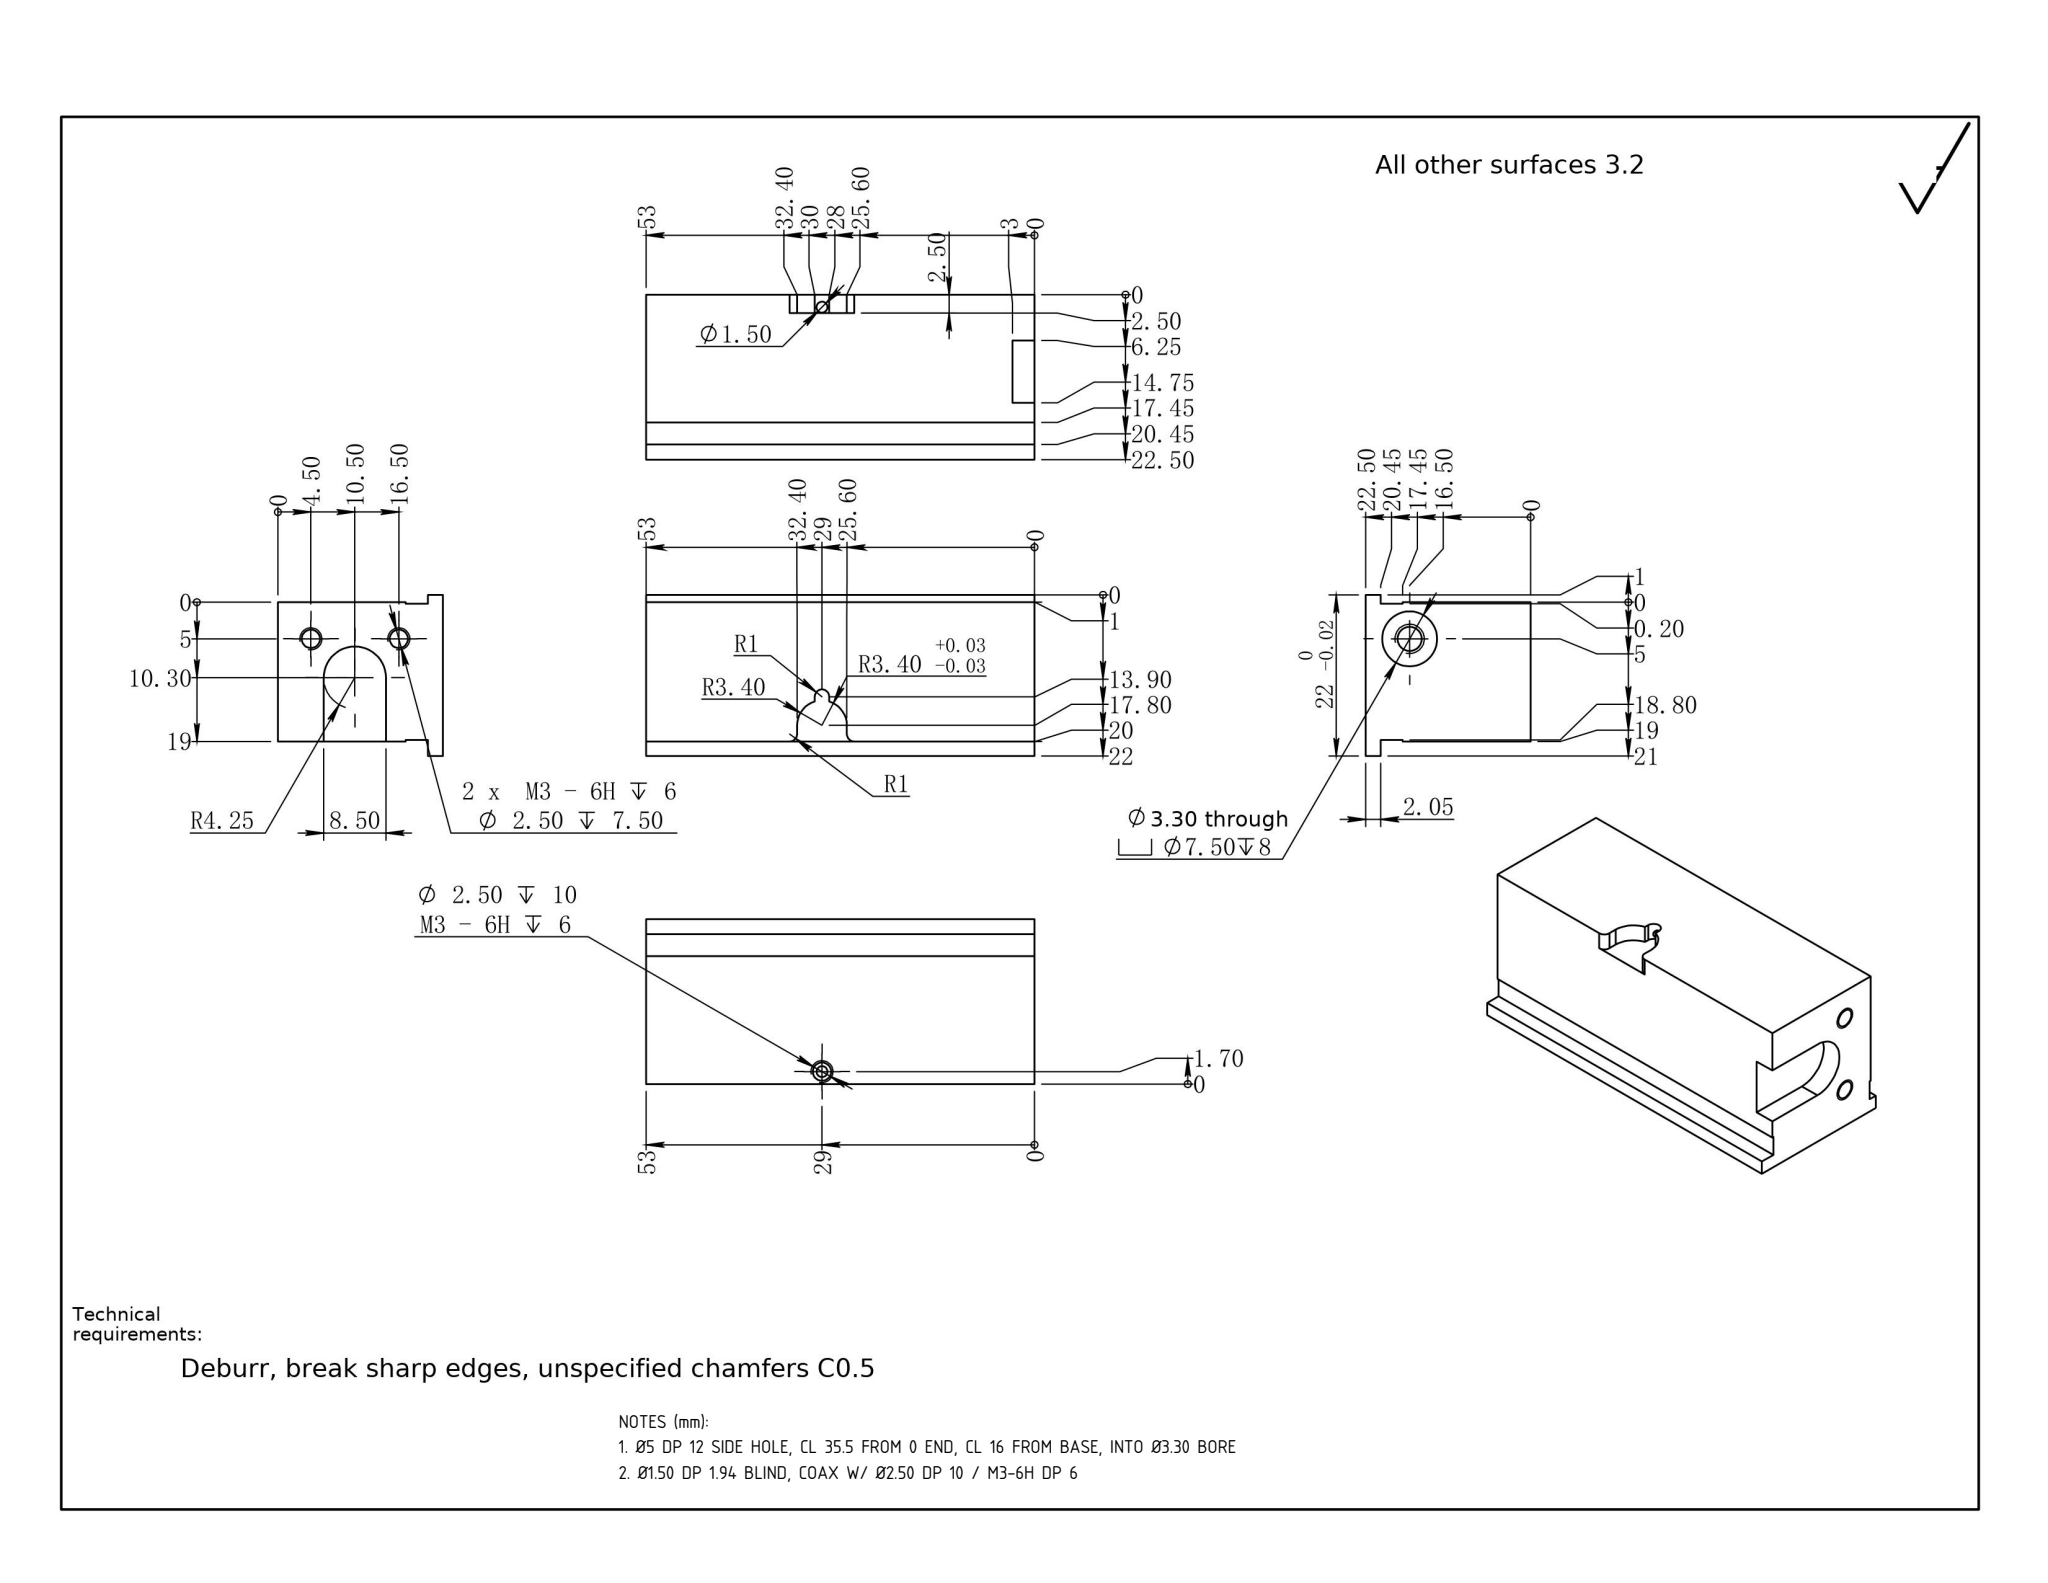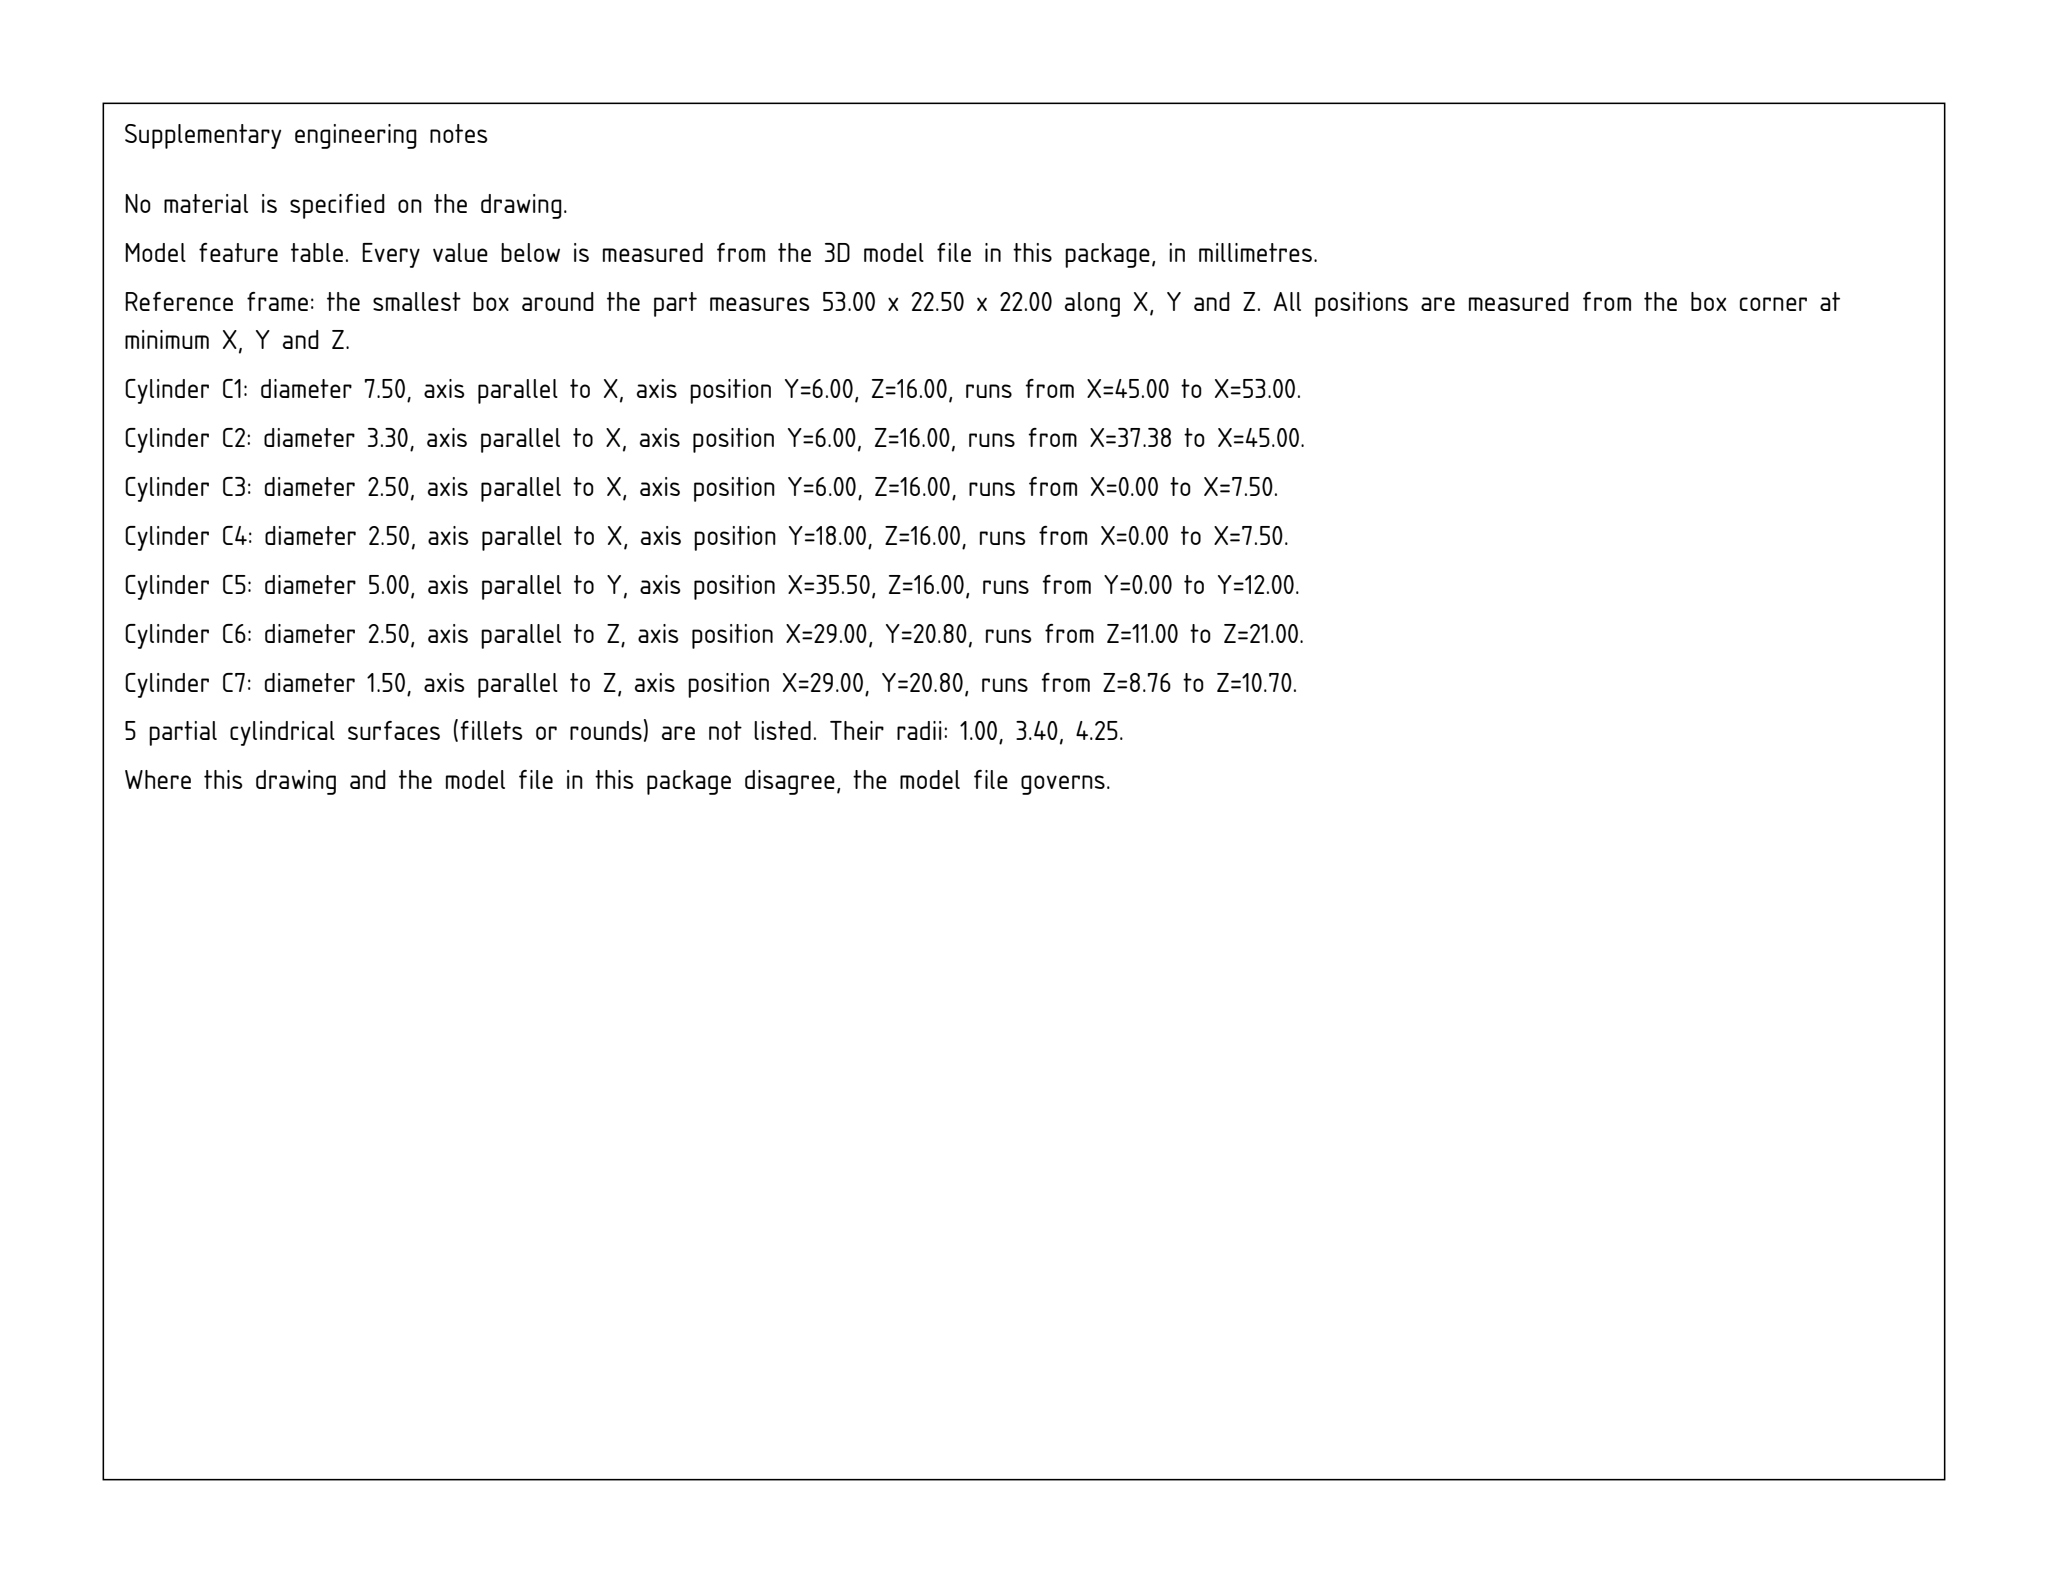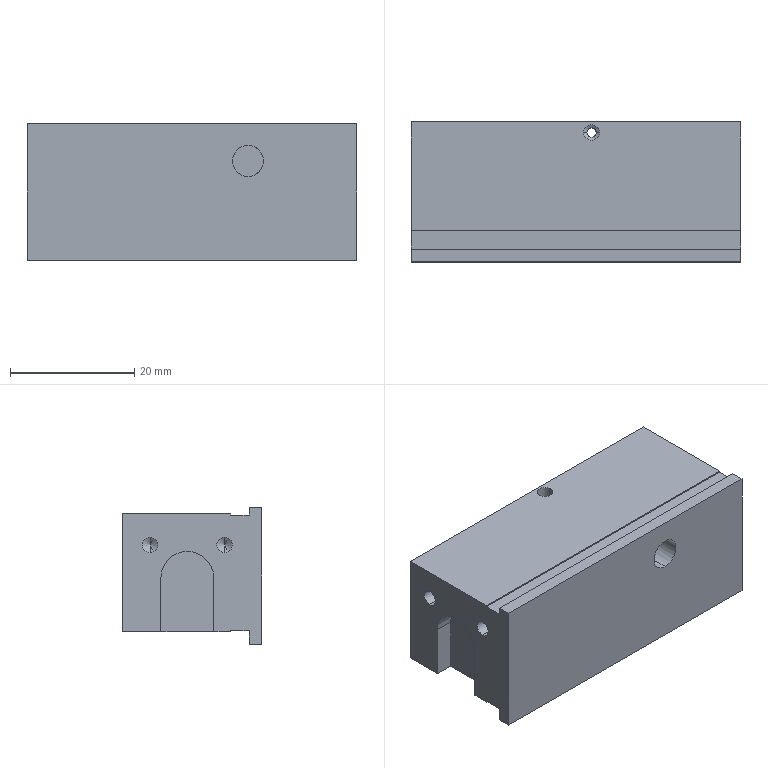Part | SolidWorks | mm | 1 solid | 51 faces | box 53 x 22.5 x 22 mm | volume 21743 mm3 | plane 24 | cylinder 21 | cone 6 | commonest cylinder face diameters 2.5 x6 2 x3 7.5 x2 3.3 x2 5 x2 8.5 x2 1.5 x2 6.8 x2
Drawing notes:
Ø5 DP 12 SIDE HOLE, CL 35.5 FROM 0 END, CL 16 FROM BASE, INTO Ø3.30 BORE | from the solid: cylinder [5.0,"y",[35.5,null,16.0],12.0]; coaxial z=16 with Ø3.30 x-bore at y=6,z=16; X datum at x=0 end face; z measured from bbox base (bbox z=22)
Ø1.50 DP 1.94 BLIND, COAX W/ Ø2.50 DP 10 / M3-6H DP 6 | from the solid: cylinders: [1.5,"z",[29.0,20.8],1.94] coaxial with [2.5,"z",[29.0,20.8],10.0]
build123d program:
from build123d import *

# Parameters (mm, degrees)
BOSS_EXTRUDE1_DEPTH        = 26.5
SKETCH25_W                 = 0.2
SKETCH25_H                 = 3
CUT_EXTRUDE12_DEPTH        = 59.62
SKETCH4_R                  = 3.4
CUT_EXTRUDE1_DEPTH         = 2.5
CUT_EXTRUDE19_DEPTH        = 3
M3_TAPPED_HOLE3_D          = 2.5
M3_TAPPED_HOLE3_DEPTH      = 7.5
M3_TAPPED_HOLE3_TIP        = 0.7511
SKETCH43_R                 = 2.5
CUT_EXTRUDE21_DEPTH        = 12
M4_TAPPED_HOLE1_D          = 3.3
M4_TAPPED_HOLE1_DEPTH      = 17.499
M4_TAPPED_HOLE1_TIP        = 0.9914
SKETCH47_W                 = 6.8
SKETCH47_H                 = 4.4
CUT_EXTRUDE22_DEPTH        = 35.975
F_1_5_1_5_DIAMETER_HOLE1_D = 1.5
M3_TAPPED_HOLE5_D          = 2.5
M3_TAPPED_HOLE5_DEPTH      = 10
M3_TAPPED_HOLE5_TIP        = 0.7511
FILLET1_R                  = 1
SKETCH54_R                 = 3.75
CUT_EXTRUDE23_DEPTH        = 8
SKETCH55_R                 = 1
SKETCH55_W                 = 2
SKETCH55_H                 = 1
CUT_EXTRUDE24_DEPTH        = 35.975


with BuildPart() as part:
    # Sketch1 → Boss-Extrude1 (new, symmetric)
    with BuildSketch(Plane(origin=(0, 0, 0), x_dir=(0, 0, -1), z_dir=(1, 0, 0))):
        Polygon((11, 0), (11, 2.05), (9, 2.05), (9, 22.5), (-10, 22.5), (-10, 2.05), (-11, 2.05), (-11, 0), align=None)
    extrude(amount=BOSS_EXTRUDE1_DEPTH, both=True)

    # Sketch25 → Cut-Extrude12 (cut, through all)
    with BuildSketch(Plane(origin=(26.5, 0, 0), x_dir=(0, 0, -1), z_dir=(1, 0, 0))):
        with Locations((-9.9, 3.55)):
            Rectangle(SKETCH25_W, SKETCH25_H)
        with Locations((8.9, 3.55)):
            Rectangle(SKETCH25_W, SKETCH25_H)
    extrude(amount=-CUT_EXTRUDE12_DEPTH, mode=Mode.SUBTRACT)

    # Sketch4 → Cut-Extrude1 (cut)
    with BuildSketch(Plane(origin=(0, 22.5, 0), x_dir=(-1, 0, 0), z_dir=(0, 1, 0))):
        with Locations((-2.5, -6.8)):
            Circle(SKETCH4_R)
    extrude(amount=-CUT_EXTRUDE1_DEPTH, mode=Mode.SUBTRACT)

    # Sketch38 → Cut-Extrude19 (cut)
    with BuildSketch(Plane(origin=(-26.5, 0, 0), x_dir=(0, 0, -1), z_dir=(1, 0, 0))):
        with BuildLine():
            Line((9, 7.75), (0.3, 7.75))
            ThreePointArc((0.3, 7.75), (-3.95, 12), (0.3, 16.25))
            Line((0.3, 16.25), (9, 16.25))
            ThreePointArc((9, 16.25), (13.25, 12), (9, 7.75))
        make_face()
    extrude(amount=CUT_EXTRUDE19_DEPTH, mode=Mode.SUBTRACT)

    # M3 Tapped Hole3
    with Locations(Plane(origin=(-26.5, 0, 0), x_dir=(0, 0, -1), z_dir=(-1, 0, 0))):
        with Locations((-5, -6), (-5, -18)):
            Hole(M3_TAPPED_HOLE3_D / 2, depth=M3_TAPPED_HOLE3_DEPTH)
            with Locations((0, 0, -(M3_TAPPED_HOLE3_DEPTH + M3_TAPPED_HOLE3_TIP / 2))):  # 118° drill point
                Cone(0, M3_TAPPED_HOLE3_D / 2, M3_TAPPED_HOLE3_TIP, mode=Mode.SUBTRACT)

    # Sketch43 → Cut-Extrude21 (cut)
    with BuildSketch(Plane.XZ):
        with Locations(Location((9, 5, 0), (0, 0, 270))):
            Circle(SKETCH43_R)
    extrude(amount=-CUT_EXTRUDE21_DEPTH, mode=Mode.SUBTRACT)

    # M4 Tapped Hole1
    with Locations(Plane(origin=(26.5, 3.474, 21.182), x_dir=(0, 0, -1), z_dir=(1, 0, 0))):
        with Locations((16.182, 2.526)):
            Hole(M4_TAPPED_HOLE1_D / 2, depth=M4_TAPPED_HOLE1_DEPTH)
            with Locations((0, 0, -(M4_TAPPED_HOLE1_DEPTH + M4_TAPPED_HOLE1_TIP / 2))):  # 118° drill point
                Cone(0, M4_TAPPED_HOLE1_D / 2, M4_TAPPED_HOLE1_TIP, mode=Mode.SUBTRACT)

    # Sketch47 → Cut-Extrude22 (cut, through all)
    with BuildSketch(Plane(origin=(0, 20, 0), x_dir=(1, 0, 0), z_dir=(0, 1, 0))):
        with Locations((2.5, 9)):
            Rectangle(SKETCH47_W, SKETCH47_H)
    extrude(amount=CUT_EXTRUDE22_DEPTH, mode=Mode.SUBTRACT)

    # 1.5 _1.5_ Diameter Hole1 (through all)
    with Locations(Plane.XY.offset(10)):
        with Locations((2.5, 20.8)):
            Hole(F_1_5_1_5_DIAMETER_HOLE1_D / 2)

    # M3 Tapped Hole5
    with Locations(Plane.XY.offset(10)):
        with Locations((2.5, 20.8)):
            Hole(M3_TAPPED_HOLE5_D / 2, depth=M3_TAPPED_HOLE5_DEPTH)
            with Locations((0, 0, -(M3_TAPPED_HOLE5_DEPTH + M3_TAPPED_HOLE5_TIP / 2))):  # 118° drill point
                Cone(0, M3_TAPPED_HOLE5_D / 2, M3_TAPPED_HOLE5_TIP, mode=Mode.SUBTRACT)

    # Fillet1
    fillet1_edges = [part.edges().sort_by_distance(p)[0] for p in [
        (5.9, 21.25, -9),
        (-0.9, 21.25, -9),
    ]]
    fillet(fillet1_edges, radius=FILLET1_R)

    # Sketch54 → Cut-Extrude23 (cut)
    with BuildSketch(Plane.ZY.offset(-26.5)):
        with Locations((5, 6)):
            Circle(SKETCH54_R)
    extrude(amount=CUT_EXTRUDE23_DEPTH, mode=Mode.SUBTRACT)

    # Sketch55 → Cut-Extrude24 (cut, through all)
    with BuildSketch(Plane(origin=(0, 20, 0), x_dir=(1, 0, 0), z_dir=(0, 1, 0))):
        with Locations((2.5, 2.9)):
            Circle(SKETCH55_R)
        with Locations((2.5, 3.4)):
            Rectangle(SKETCH55_W, SKETCH55_H)
    extrude(amount=CUT_EXTRUDE24_DEPTH, mode=Mode.SUBTRACT)


solid = part.part